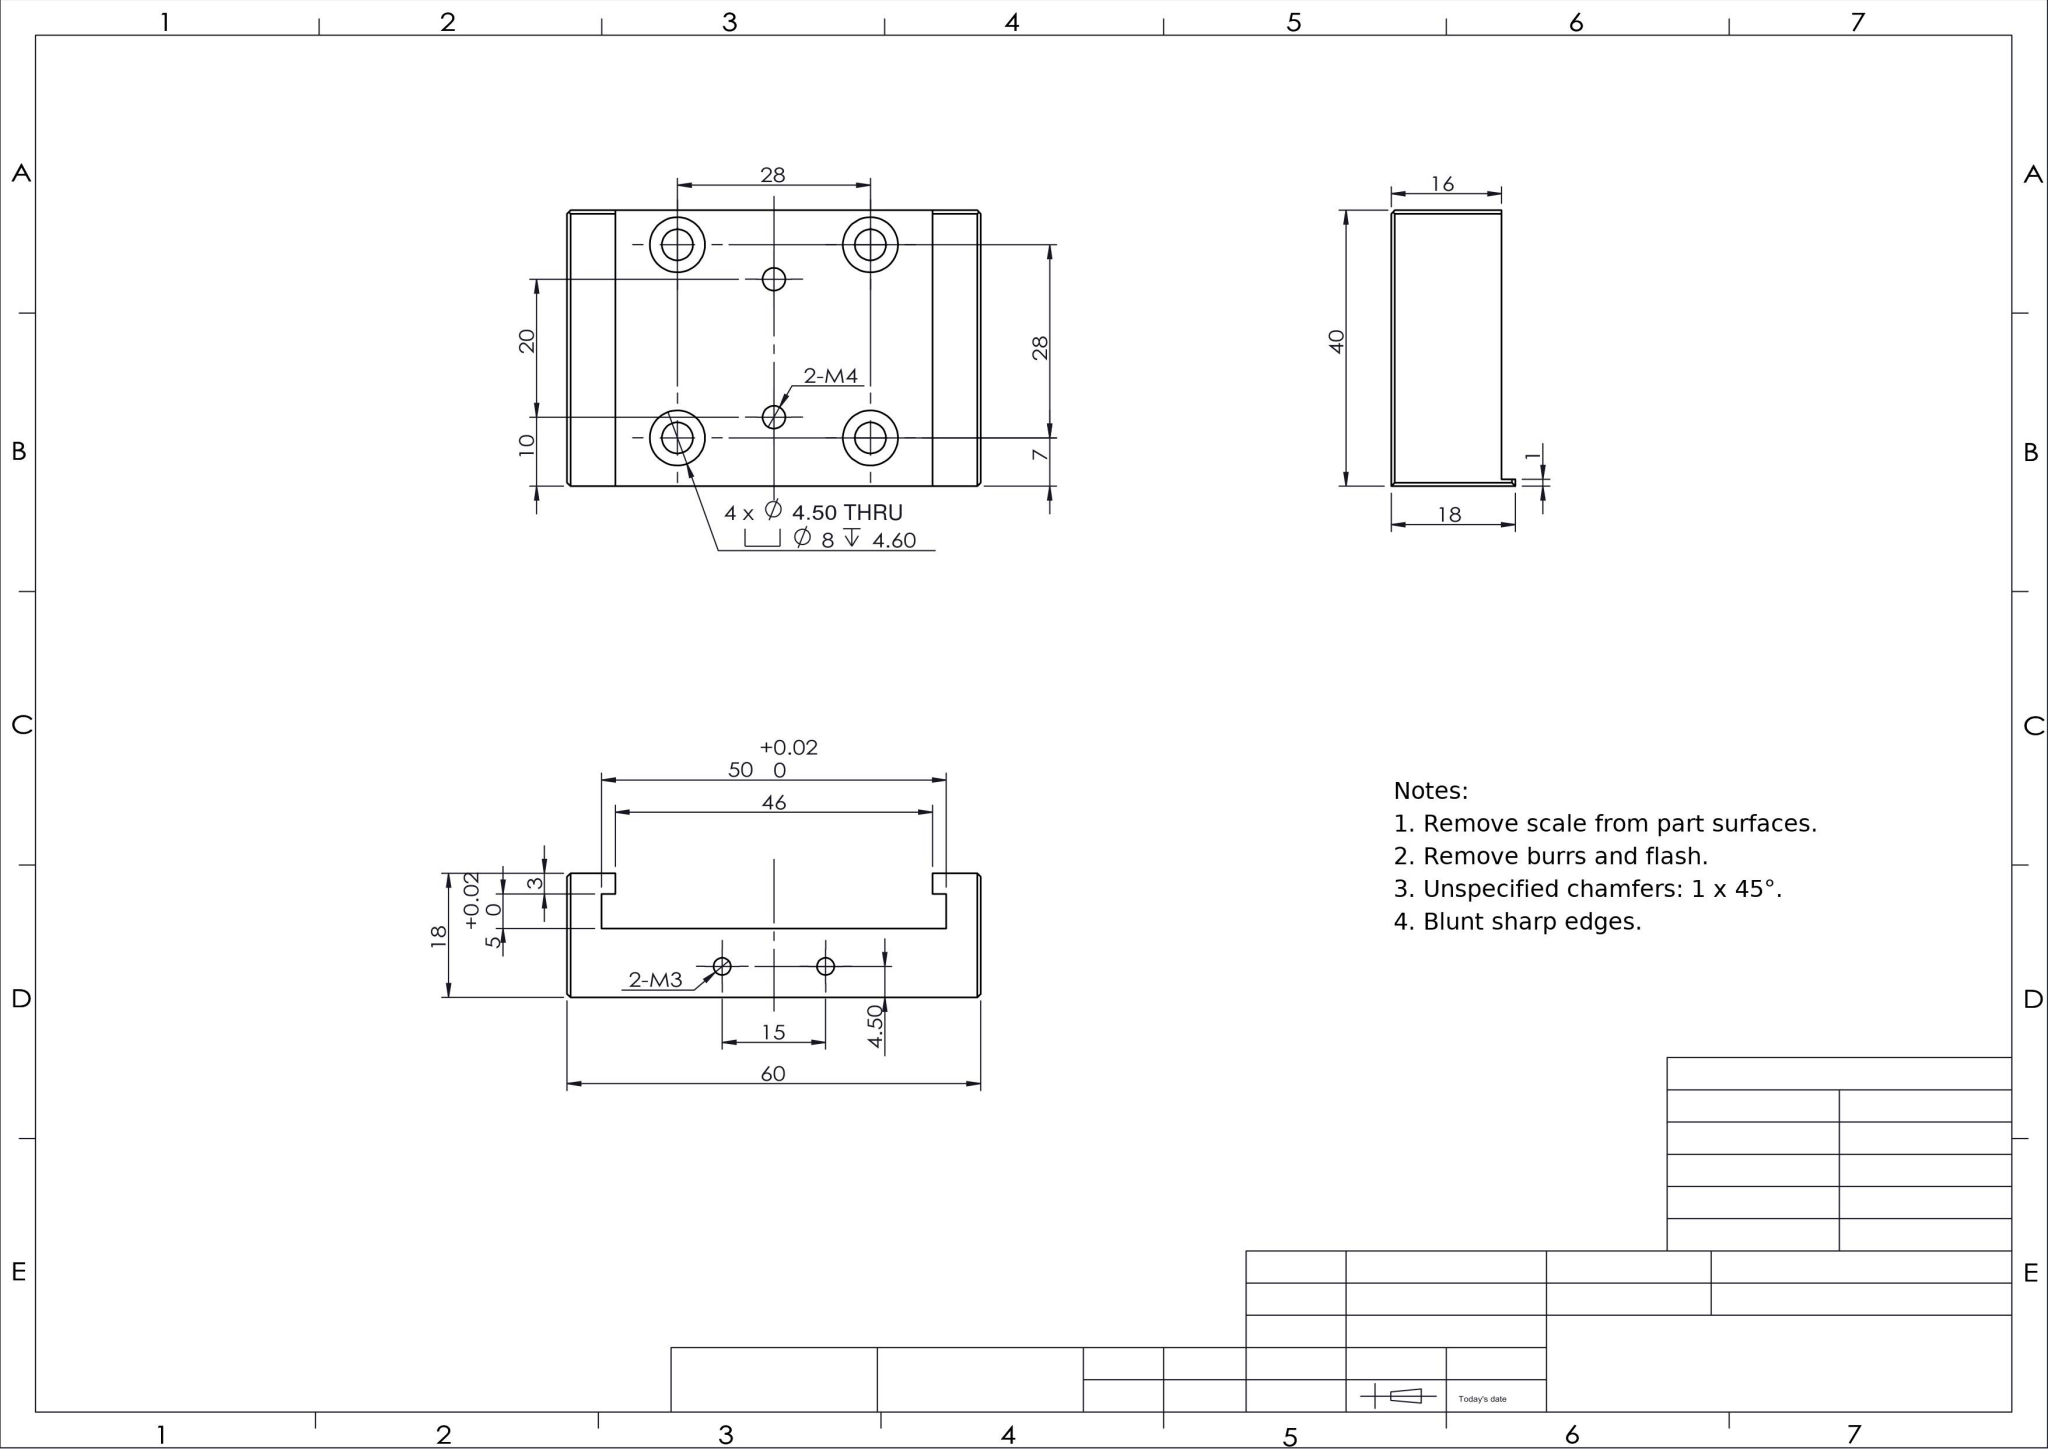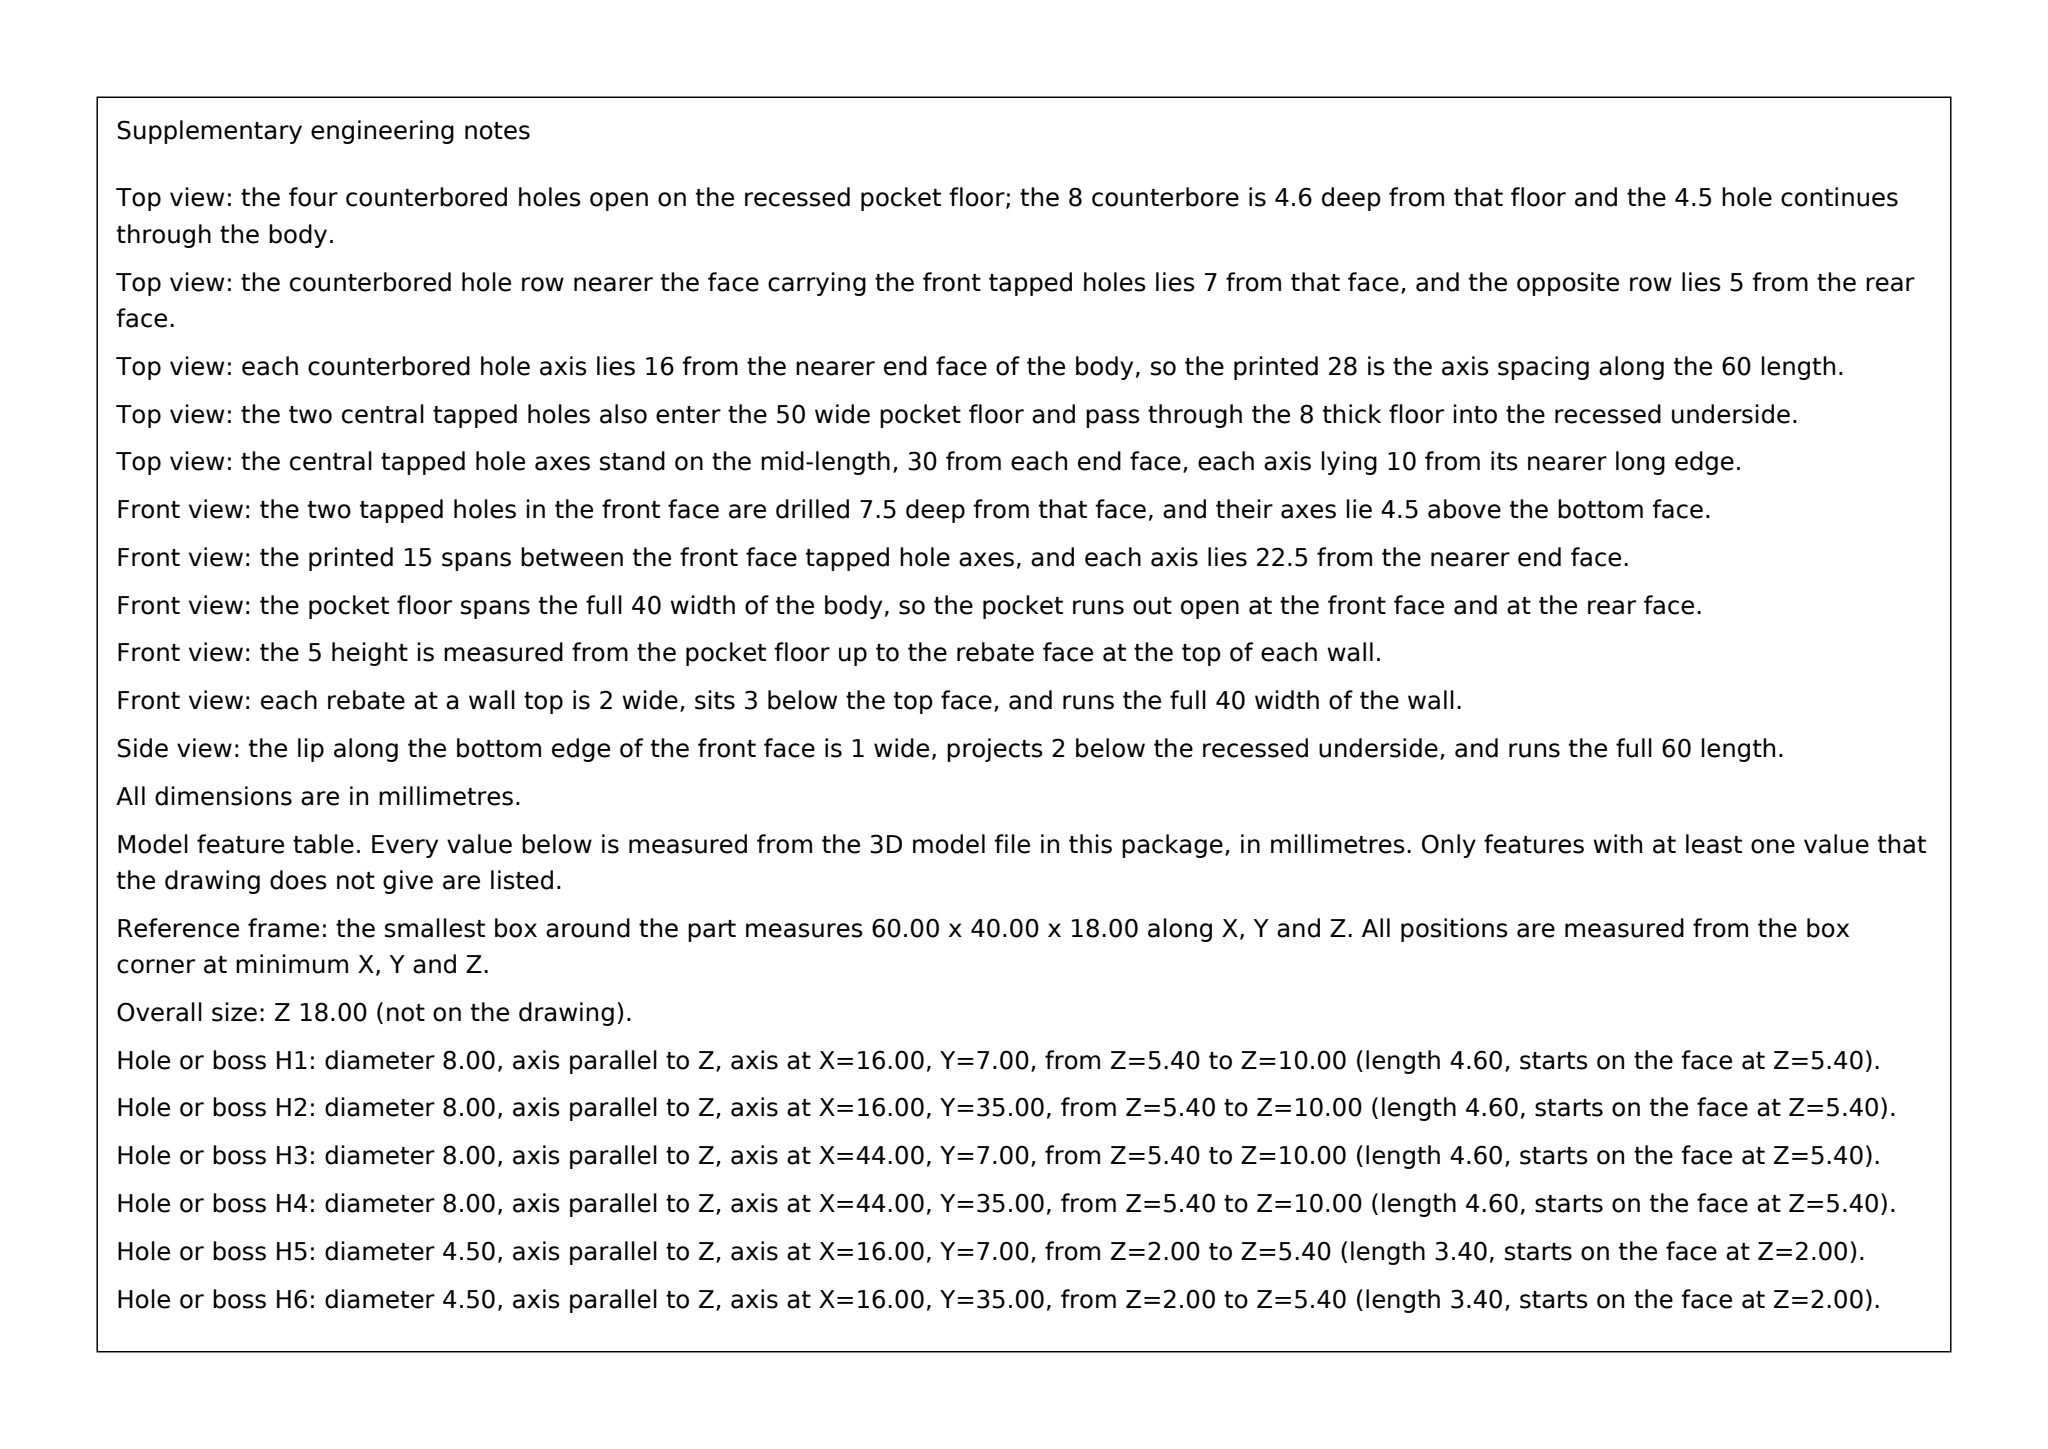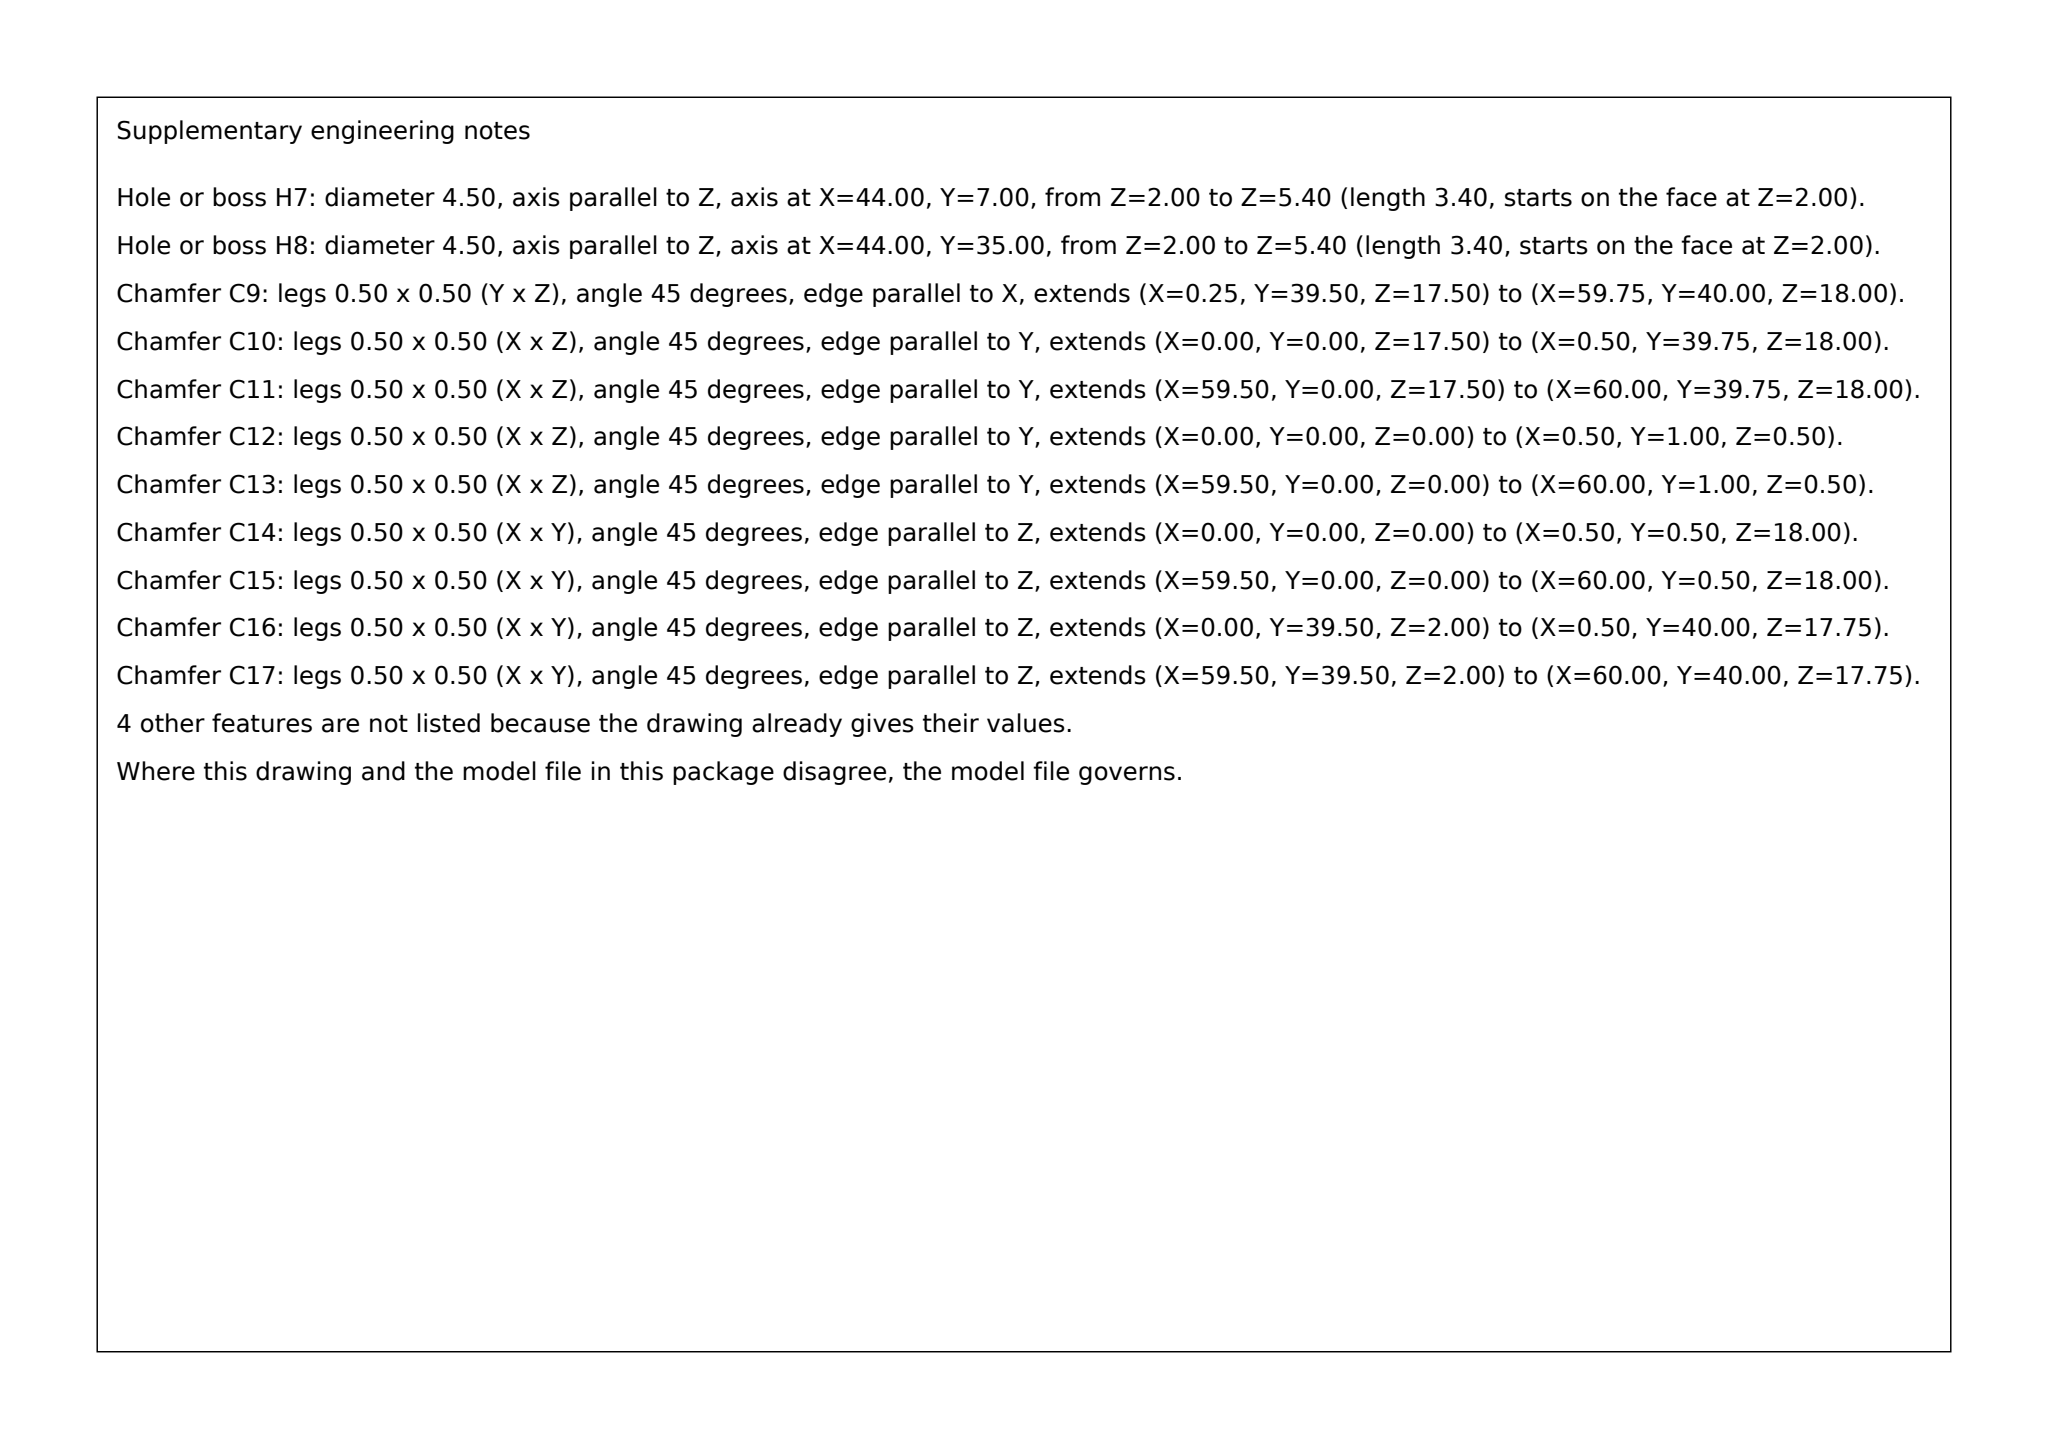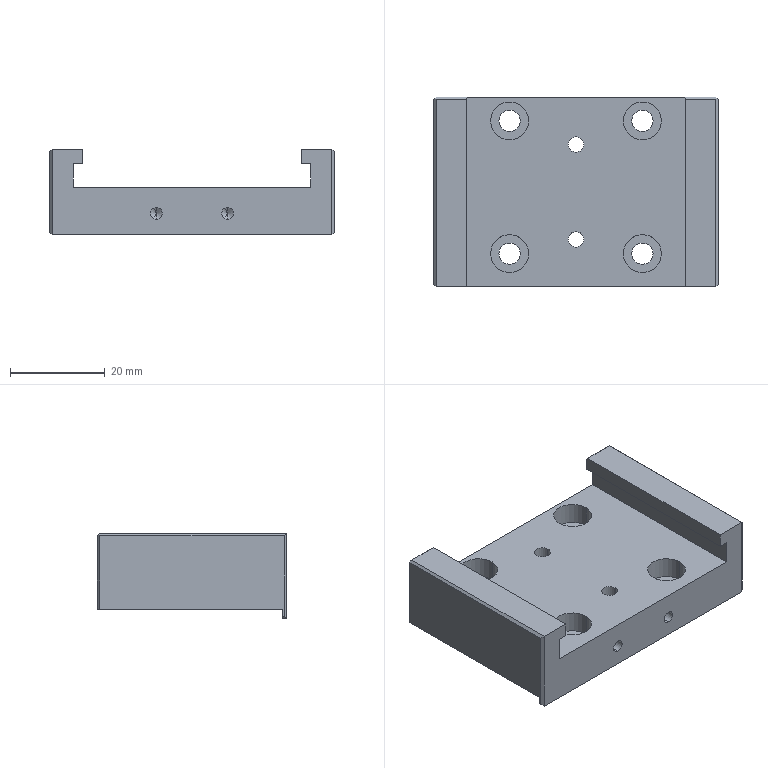Part | SolidWorks | mm | 1 solid | 58 faces | box 60 x 40 x 18 mm | volume 21626 mm3 | plane 30 | cylinder 24 | cone 4 | commonest cylinder face diameters 8 x8 4.5 x8 2.5 x4 3.3 x4
Drawing notes:
46 W SLOT 8 DP FROM TOP FACE, THRU FULL 40 WIDTH | from the solid: x planes 7/53 (46 W), z 18 top to z 10 floor = 8 DP; only y planes 0,1,40 -> no end faces
50 W CNR RELIEF 3 DP FROM TOP FACE, THRU FULL 40 WIDTH | from the solid: x planes 5/55 (50 W), z 18 to z 15 = 3 DP; no y end faces -> runs full 40
2-M4 THRU SLOT FLOOR (8 THK) ON 60 CL, 10 & 30 FROM M3 FACE, TAP FULL DP | from the solid: Ø3.3 z-axis cyls at (30,10) & (30,30), length 8.0 = floor z=2 to z=10, no drill cone
build123d program:
from build123d import *

# Parameters (mm, degrees)
SKETCH1_W                                            = 60
SKETCH1_H                                            = 40
BOSS_EXTRUDE1_DEPTH                                  = 18
SKETCH2_W                                            = 80.022
SKETCH2_H                                            = 40
CUT_EXTRUDE1_DEPTH                                   = 2
SKETCH3_W                                            = 46
SKETCH3_H                                            = 119.729
CUT_EXTRUDE2_DEPTH                                   = 8
HOLE_SIZE_ACCORDING_TO_THE_TYPE_OF_HEXAG_D           = 4.5
HOLE_SIZE_ACCORDING_TO_THE_TYPE_OF_HEXAG_CBORE_D     = 8
HOLE_SIZE_ACCORDING_TO_THE_TYPE_OF_HEXAG_CBORE_DEPTH = 4.6
M4_TAPPED_HOLE2_D                                    = 3.3
M4_TAPPED_HOLE2_DEPTH                                = 10.1
M4_TAPPED_HOLE2_TIP                                  = 0.9914
SKETCH10_W                                           = 50
SKETCH10_H                                           = 5
CUT_EXTRUDE3_DEPTH                                   = 75.324
CHAMFER1_SIZE                                        = 0.5
CHAMFER2_SIZE                                        = 0.5
CHAMFER3_SIZE                                        = 0.5
CHAMFER4_SIZE                                        = 0.5
M3_TAPPED_HOLE1_D                                    = 2.5
M3_TAPPED_HOLE1_DEPTH                                = 7.5
M3_TAPPED_HOLE1_TIP                                  = 0.7511


with BuildPart() as part:
    # Sketch1 → Boss-Extrude1 (new body)
    with BuildSketch(Plane.XY):
        with Locations((30, 20)):
            Rectangle(SKETCH1_W, SKETCH1_H)
    extrude(amount=BOSS_EXTRUDE1_DEPTH)

    # Sketch2 → Cut-Extrude1 (cut)
    with BuildSketch(Plane(origin=(0, 0, 0), x_dir=(-1, 0, 0), z_dir=(0, 0, -1))):
        with Locations((-30, 21)):
            Rectangle(SKETCH2_W, SKETCH2_H)
    extrude(amount=-CUT_EXTRUDE1_DEPTH, mode=Mode.SUBTRACT)

    # Sketch3 → Cut-Extrude2 (cut)
    with BuildSketch(Plane.XY.offset(18)):
        with Locations((30, 33.235)):
            Rectangle(SKETCH3_W, SKETCH3_H)
    extrude(amount=-CUT_EXTRUDE2_DEPTH, mode=Mode.SUBTRACT)

    # Hole Size according to the type of Hexag (through all)
    with Locations(Plane.XY.offset(10)):
        with Locations((44, 7), (16, 7), (44, 35), (16, 35)):
            CounterBoreHole(HOLE_SIZE_ACCORDING_TO_THE_TYPE_OF_HEXAG_D / 2, HOLE_SIZE_ACCORDING_TO_THE_TYPE_OF_HEXAG_CBORE_D / 2, HOLE_SIZE_ACCORDING_TO_THE_TYPE_OF_HEXAG_CBORE_DEPTH)

    # M4 Tapped Hole2
    with Locations(Plane.XY.offset(10)):
        with Locations((30, 10), (30, 30)):
            Hole(M4_TAPPED_HOLE2_D / 2, depth=M4_TAPPED_HOLE2_DEPTH)
            with Locations((0, 0, -(M4_TAPPED_HOLE2_DEPTH + M4_TAPPED_HOLE2_TIP / 2))):  # 118° drill point
                Cone(0, M4_TAPPED_HOLE2_D / 2, M4_TAPPED_HOLE2_TIP, mode=Mode.SUBTRACT)

    # Sketch10 → Cut-Extrude3 (cut, through all)
    with BuildSketch(Plane.XZ):
        with Locations((30, 12.5)):
            Rectangle(SKETCH10_W, SKETCH10_H)
    extrude(amount=-CUT_EXTRUDE3_DEPTH, mode=Mode.SUBTRACT)

    # Chamfer1
    chamfer1_edges = [part.edges().sort_by_distance(p)[0] for p in [
        (60, 0, 9),
        (0, 0, 9),
        (0, 40, 10),
        (60, 40, 10),
    ]]
    chamfer(chamfer1_edges, length=CHAMFER1_SIZE)

    # Chamfer2
    chamfer2_edges = [part.edges().sort_by_distance(p)[0] for p in [
        (0, 20, 18),
        (60, 20, 18),
    ]]
    chamfer(chamfer2_edges, length=CHAMFER2_SIZE)

    # Chamfer3
    chamfer3_edges = [part.edges().sort_by_distance(p)[0] for p in [
        (0, 0.75, 0),
        (60, 0.75, 0),
    ]]
    chamfer(chamfer3_edges, length=CHAMFER3_SIZE)

    # Chamfer4
    chamfer4_edges = [part.edges().sort_by_distance(p)[0] for p in [
        (56.25, 40, 18),
        (3.75, 40, 18),
    ]]
    chamfer(chamfer4_edges, length=CHAMFER4_SIZE)

    # M3 Tapped Hole1
    with Locations(Plane(origin=(0, 0, 0), x_dir=(-1, 0, 0), z_dir=(0, -1, 0))):
        with Locations((-22.5, -4.5), (-37.5, -4.5)):
            Hole(M3_TAPPED_HOLE1_D / 2, depth=M3_TAPPED_HOLE1_DEPTH)
            with Locations((0, 0, -(M3_TAPPED_HOLE1_DEPTH + M3_TAPPED_HOLE1_TIP / 2))):  # 118° drill point
                Cone(0, M3_TAPPED_HOLE1_D / 2, M3_TAPPED_HOLE1_TIP, mode=Mode.SUBTRACT)


solid = part.part